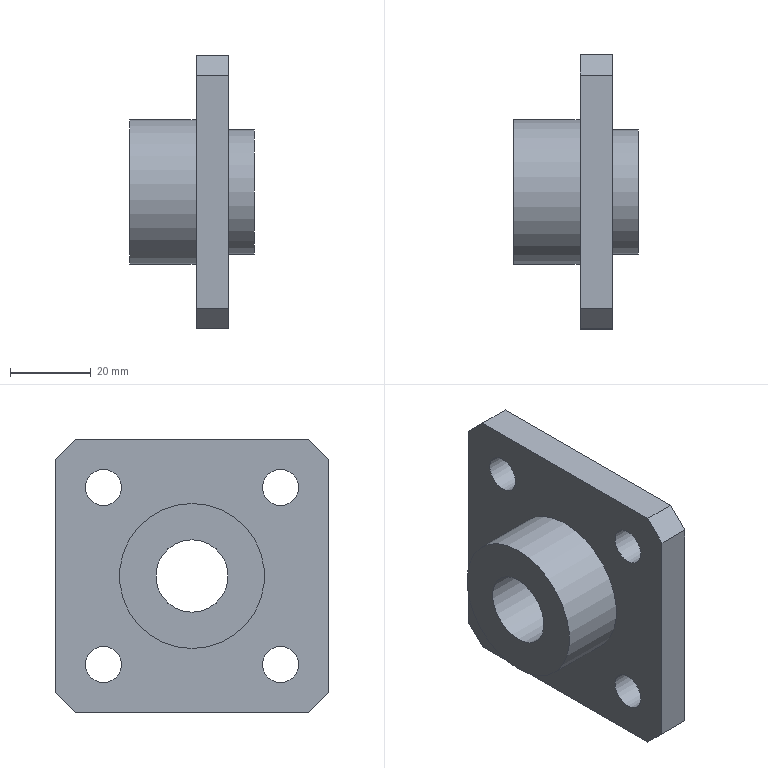Component | NX | END_CAP | 1 solid | 19 faces | volume 48369 mm3 | plane 12 | cylinder 7 | commonest cylinder face diameters 9 x4 18 x1 31 x1 36 x1